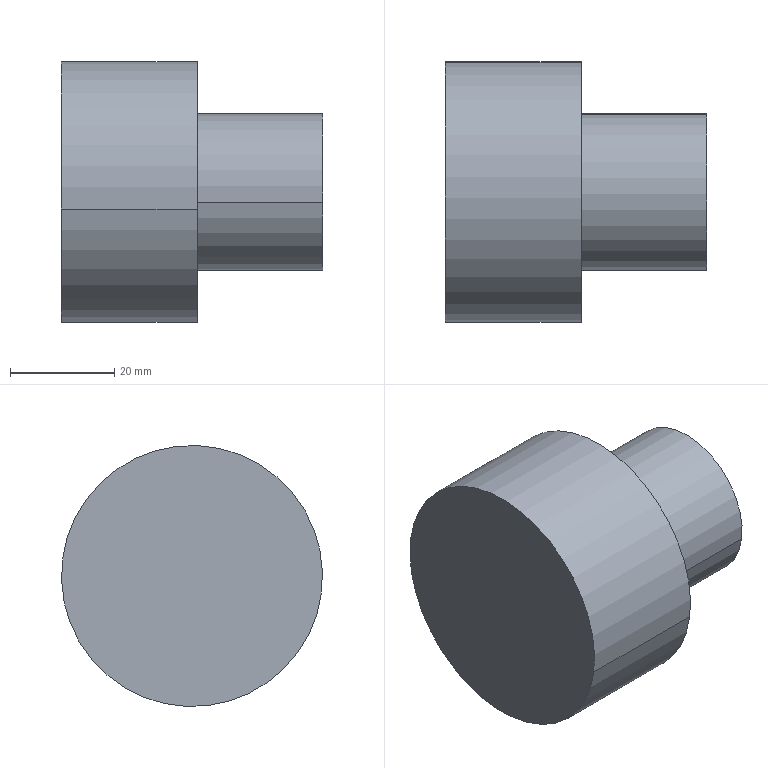Component | SolidWorks | -BeltTensionHandwheel-1 | 1 solid | 10 faces | box 50 x 50 x 50 mm | volume 66319 mm3 | cylinder 6 | plane 4 | commonest cylinder face diameters 12 x2 30 x2 50 x2
build123d program:
from build123d import *


with BuildPart() as part:
    # Sketch1 → Revolve1 (revolve)
    with BuildSketch(Plane.XY):
        Polygon((0, 0), (25, 0), (25, 26), (15, 26), (15, 50), (6, 50), (6, 35), (0, 35), align=None)
    revolve(axis=Axis((0, -469.095, 0), (0, 1, 0)))


solid = part.part

# Placed as in the assembly
solid = solid.moved(Location((-325, 1094.5, -20), (0, 0, -90)))
STEP:
#1=COLOUR_RGB('',0.7922,0.8196,0.9333);
#2=FILL_AREA_STYLE_COLOUR('',#1);
#3=FILL_AREA_STYLE('',(#2));
#4=SURFACE_STYLE_FILL_AREA(#3);
#5=SURFACE_SIDE_STYLE('',(#4));
#6=SURFACE_STYLE_USAGE(.BOTH.,#5);
#7=PRESENTATION_STYLE_ASSIGNMENT((#6));
#8=CARTESIAN_POINT('',(-10.827,43.325,-0.7566));
#9=VERTEX_POINT('',#8);
#10=CARTESIAN_POINT('',(-10.827,42.856,-0.8182));
#11=VERTEX_POINT('',#10);
#12=CARTESIAN_POINT('',(-10.827,43.091,-0.7874));
#13=DIRECTION('',(-1.,0.,-0.));
#14=DIRECTION('',(-0.,-0.9915,-0.1304));
#15=AXIS2_PLACEMENT_3D('',#12,#13,#14);
#16=CIRCLE('',#15,0.2362);
#17=EDGE_CURVE('',#9,#11,#16,.T.);
#18=ORIENTED_EDGE('',*,*,#17,.F.);
#19=CARTESIAN_POINT('',(-11.417,43.325,-0.7566));
#20=VERTEX_POINT('',#19);
#21=CARTESIAN_POINT('',(-31.264,43.325,-0.7566));
#22=DIRECTION('',(-1.,0.,-0.));
#23=VECTOR('',#22,39.37);
#24=LINE('',#21,#23);
#25=EDGE_CURVE('',#9,#20,#24,.T.);
#26=ORIENTED_EDGE('',*,*,#25,.T.);
#27=CARTESIAN_POINT('',(-11.417,42.856,-0.8182));
#28=VERTEX_POINT('',#27);
#29=CARTESIAN_POINT('',(-11.417,43.091,-0.7874));
#30=DIRECTION('',(-1.,0.,-0.));
#31=DIRECTION('',(-0.,-0.9915,-0.1304));
#32=AXIS2_PLACEMENT_3D('',#29,#30,#31);
#33=CIRCLE('',#32,0.2362);
#34=EDGE_CURVE('',#20,#28,#33,.T.);
#35=ORIENTED_EDGE('',*,*,#34,.T.);
#36=CARTESIAN_POINT('',(-31.264,42.856,-0.8182));
#37=DIRECTION('',(-1.,0.,-0.));
#38=VECTOR('',#37,39.37);
#39=LINE('',#36,#38);
#40=EDGE_CURVE('',#11,#28,#39,.T.);
#41=ORIENTED_EDGE('',*,*,#40,.F.);
#42=EDGE_LOOP('',(#18,#26,#35,#41));
#43=FACE_OUTER_BOUND('',#42,.T.);
#44=CARTESIAN_POINT('',(-31.264,43.091,-0.7874));
#45=DIRECTION('',(-1.,0.,-0.));
#46=DIRECTION('',(-0.,-0.9915,-0.1304));
#47=AXIS2_PLACEMENT_3D('',#44,#45,#46);
#48=CYLINDRICAL_SURFACE('',#47,0.2362);
#49=ADVANCED_FACE('',(#43),#48,.F.);
#50=CARTESIAN_POINT('',(-10.827,42.505,-0.8644));
#51=VERTEX_POINT('',#50);
#52=CARTESIAN_POINT('',(-10.827,43.676,-0.7104));
#53=VERTEX_POINT('',#52);
#54=CARTESIAN_POINT('',(-10.827,43.091,-0.7874));
#55=DIRECTION('',(-1.,0.,-0.));
#56=DIRECTION('',(-0.,-0.9915,-0.1304));
#57=AXIS2_PLACEMENT_3D('',#54,#55,#56);
#58=CIRCLE('',#57,0.5906);
#59=EDGE_CURVE('',#51,#53,#58,.T.);
#60=ORIENTED_EDGE('',*,*,#59,.T.);
#61=CARTESIAN_POINT('',(-11.772,43.676,-0.7104));
#62=VERTEX_POINT('',#61);
#63=CARTESIAN_POINT('',(-31.264,43.676,-0.7104));
#64=DIRECTION('',(-1.,0.,-0.));
#65=VECTOR('',#64,39.37);
#66=LINE('',#63,#65);
#67=EDGE_CURVE('',#53,#62,#66,.T.);
#68=ORIENTED_EDGE('',*,*,#67,.T.);
#69=CARTESIAN_POINT('',(-11.772,42.505,-0.8644));
#70=VERTEX_POINT('',#69);
#71=CARTESIAN_POINT('',(-11.772,43.091,-0.7874));
#72=DIRECTION('',(-1.,0.,-0.));
#73=DIRECTION('',(-0.,-0.9915,-0.1304));
#74=AXIS2_PLACEMENT_3D('',#71,#72,#73);
#75=CIRCLE('',#74,0.5906);
#76=EDGE_CURVE('',#70,#62,#75,.T.);
#77=ORIENTED_EDGE('',*,*,#76,.F.);
#78=CARTESIAN_POINT('',(-31.264,42.505,-0.8644));
#79=DIRECTION('',(-1.,0.,-0.));
#80=VECTOR('',#79,39.37);
#81=LINE('',#78,#80);
#82=EDGE_CURVE('',#51,#70,#81,.T.);
#83=ORIENTED_EDGE('',*,*,#82,.F.);
#84=EDGE_LOOP('',(#60,#68,#77,#83));
#85=FACE_OUTER_BOUND('',#84,.T.);
#86=CARTESIAN_POINT('',(-31.264,43.091,-0.7874));
#87=DIRECTION('',(-1.,0.,-0.));
#88=DIRECTION('',(-0.,-0.9915,-0.1304));
#89=AXIS2_PLACEMENT_3D('',#86,#87,#88);
#90=CYLINDRICAL_SURFACE('',#89,0.5906);
#91=ADVANCED_FACE('',(#85),#90,.T.);
#92=CARTESIAN_POINT('',(-11.772,42.115,-0.9158));
#93=VERTEX_POINT('',#92);
#94=CARTESIAN_POINT('',(-11.772,44.066,-0.659));
#95=VERTEX_POINT('',#94);
#96=CARTESIAN_POINT('',(-11.772,43.091,-0.7874));
#97=DIRECTION('',(-1.,0.,-0.));
#98=DIRECTION('',(-0.,-0.9915,-0.1304));
#99=AXIS2_PLACEMENT_3D('',#96,#97,#98);
#100=CIRCLE('',#99,0.9843);
#101=EDGE_CURVE('',#93,#95,#100,.T.);
#102=ORIENTED_EDGE('',*,*,#101,.T.);
#103=CARTESIAN_POINT('',(-12.795,44.066,-0.659));
#104=VERTEX_POINT('',#103);
#105=CARTESIAN_POINT('',(-31.264,44.066,-0.659));
#106=DIRECTION('',(-1.,0.,-0.));
#107=VECTOR('',#106,39.37);
#108=LINE('',#105,#107);
#109=EDGE_CURVE('',#95,#104,#108,.T.);
#110=ORIENTED_EDGE('',*,*,#109,.T.);
#111=CARTESIAN_POINT('',(-12.795,42.115,-0.9158));
#112=VERTEX_POINT('',#111);
#113=CARTESIAN_POINT('',(-12.795,43.091,-0.7874));
#114=DIRECTION('',(-1.,0.,-0.));
#115=DIRECTION('',(-0.,-0.9915,-0.1304));
#116=AXIS2_PLACEMENT_3D('',#113,#114,#115);
#117=CIRCLE('',#116,0.9843);
#118=EDGE_CURVE('',#112,#104,#117,.T.);
#119=ORIENTED_EDGE('',*,*,#118,.F.);
#120=CARTESIAN_POINT('',(-31.264,42.115,-0.9158));
#121=DIRECTION('',(-1.,0.,-0.));
#122=VECTOR('',#121,39.37);
#123=LINE('',#120,#122);
#124=EDGE_CURVE('',#93,#112,#123,.T.);
#125=ORIENTED_EDGE('',*,*,#124,.F.);
#126=EDGE_LOOP('',(#102,#110,#119,#125));
#127=FACE_OUTER_BOUND('',#126,.T.);
#128=CARTESIAN_POINT('',(-31.264,43.091,-0.7874));
#129=DIRECTION('',(-1.,0.,-0.));
#130=DIRECTION('',(-0.,-0.9915,-0.1304));
#131=AXIS2_PLACEMENT_3D('',#128,#129,#130);
#132=CYLINDRICAL_SURFACE('',#131,0.9843);
#133=ADVANCED_FACE('',(#127),#132,.T.);
#134=ORIENTED_EDGE('',*,*,#118,.T.);
#135=CARTESIAN_POINT('',(-12.795,43.091,-0.7874));
#136=DIRECTION('',(-1.,0.,-0.));
#137=DIRECTION('',(-0.,-0.9915,-0.1304));
#138=AXIS2_PLACEMENT_3D('',#135,#136,#137);
#139=CIRCLE('',#138,0.9843);
#140=EDGE_CURVE('',#104,#112,#139,.T.);
#141=ORIENTED_EDGE('',*,*,#140,.T.);
#142=EDGE_LOOP('',(#134,#141));
#143=FACE_OUTER_BOUND('',#142,.T.);
#144=CARTESIAN_POINT('',(-12.795,43.091,-0.7874));
#145=DIRECTION('',(-1.,0.,-0.));
#146=DIRECTION('',(-0.,-0.9915,-0.1304));
#147=AXIS2_PLACEMENT_3D('',#144,#145,#146);
#148=PLANE('',#147);
#149=ADVANCED_FACE('',(#143),#148,.T.);
#150=ORIENTED_EDGE('',*,*,#109,.F.);
#151=CARTESIAN_POINT('',(-11.772,43.091,-0.7874));
#152=DIRECTION('',(-1.,0.,-0.));
#153=DIRECTION('',(-0.,-0.9915,-0.1304));
#154=AXIS2_PLACEMENT_3D('',#151,#152,#153);
#155=CIRCLE('',#154,0.9843);
#156=EDGE_CURVE('',#95,#93,#155,.T.);
#157=ORIENTED_EDGE('',*,*,#156,.T.);
#158=ORIENTED_EDGE('',*,*,#124,.T.);
#159=ORIENTED_EDGE('',*,*,#140,.F.);
#160=EDGE_LOOP('',(#150,#157,#158,#159));
#161=FACE_OUTER_BOUND('',#160,.T.);
#162=CARTESIAN_POINT('',(-31.264,43.091,-0.7874));
#163=DIRECTION('',(-1.,0.,-0.));
#164=DIRECTION('',(-0.,-0.9915,-0.1304));
#165=AXIS2_PLACEMENT_3D('',#162,#163,#164);
#166=CYLINDRICAL_SURFACE('',#165,0.9843);
#167=ADVANCED_FACE('',(#161),#166,.T.);
#168=ORIENTED_EDGE('',*,*,#76,.T.);
#169=CARTESIAN_POINT('',(-11.772,43.091,-0.7874));
#170=DIRECTION('',(-1.,0.,-0.));
#171=DIRECTION('',(-0.,-0.9915,-0.1304));
#172=AXIS2_PLACEMENT_3D('',#169,#170,#171);
#173=CIRCLE('',#172,0.5906);
#174=EDGE_CURVE('',#62,#70,#173,.T.);
#175=ORIENTED_EDGE('',*,*,#174,.T.);
#176=EDGE_LOOP('',(#168,#175));
#177=FACE_BOUND('',#176,.T.);
#178=ORIENTED_EDGE('',*,*,#101,.F.);
#179=ORIENTED_EDGE('',*,*,#156,.F.);
#180=EDGE_LOOP('',(#178,#179));
#181=FACE_OUTER_BOUND('',#180,.T.);
#182=CARTESIAN_POINT('',(-11.772,42.115,-0.9158));
#183=DIRECTION('',(1.,-0.,0.));
#184=DIRECTION('',(0.,0.9915,0.1304));
#185=AXIS2_PLACEMENT_3D('',#182,#183,#184);
#186=PLANE('',#185);
#187=ADVANCED_FACE('',(#177,#181),#186,.T.);
#188=ORIENTED_EDGE('',*,*,#67,.F.);
#189=CARTESIAN_POINT('',(-10.827,43.091,-0.7874));
#190=DIRECTION('',(-1.,0.,-0.));
#191=DIRECTION('',(-0.,-0.9915,-0.1304));
#192=AXIS2_PLACEMENT_3D('',#189,#190,#191);
#193=CIRCLE('',#192,0.5906);
#194=EDGE_CURVE('',#53,#51,#193,.T.);
#195=ORIENTED_EDGE('',*,*,#194,.T.);
#196=ORIENTED_EDGE('',*,*,#82,.T.);
#197=ORIENTED_EDGE('',*,*,#174,.F.);
#198=EDGE_LOOP('',(#188,#195,#196,#197));
#199=FACE_OUTER_BOUND('',#198,.T.);
#200=CARTESIAN_POINT('',(-31.264,43.091,-0.7874));
#201=DIRECTION('',(-1.,0.,-0.));
#202=DIRECTION('',(-0.,-0.9915,-0.1304));
#203=AXIS2_PLACEMENT_3D('',#200,#201,#202);
#204=CYLINDRICAL_SURFACE('',#203,0.5906);
#205=ADVANCED_FACE('',(#199),#204,.T.);
#206=CARTESIAN_POINT('',(-10.827,43.091,-0.7874));
#207=DIRECTION('',(-1.,0.,-0.));
#208=DIRECTION('',(-0.,-0.9915,-0.1304));
#209=AXIS2_PLACEMENT_3D('',#206,#207,#208);
#210=CIRCLE('',#209,0.2362);
#211=EDGE_CURVE('',#11,#9,#210,.T.);
#212=ORIENTED_EDGE('',*,*,#211,.T.);
#213=ORIENTED_EDGE('',*,*,#17,.T.);
#214=EDGE_LOOP('',(#212,#213));
#215=FACE_BOUND('',#214,.T.);
#216=ORIENTED_EDGE('',*,*,#59,.F.);
#217=ORIENTED_EDGE('',*,*,#194,.F.);
#218=EDGE_LOOP('',(#216,#217));
#219=FACE_OUTER_BOUND('',#218,.T.);
#220=CARTESIAN_POINT('',(-10.827,42.505,-0.8644));
#221=DIRECTION('',(1.,-0.,0.));
#222=DIRECTION('',(0.,0.9915,0.1304));
#223=AXIS2_PLACEMENT_3D('',#220,#221,#222);
#224=PLANE('',#223);
#225=ADVANCED_FACE('',(#215,#219),#224,.T.);
#226=ORIENTED_EDGE('',*,*,#25,.F.);
#227=ORIENTED_EDGE('',*,*,#211,.F.);
#228=ORIENTED_EDGE('',*,*,#40,.T.);
#229=CARTESIAN_POINT('',(-11.417,43.091,-0.7874));
#230=DIRECTION('',(-1.,0.,-0.));
#231=DIRECTION('',(-0.,-0.9915,-0.1304));
#232=AXIS2_PLACEMENT_3D('',#229,#230,#231);
#233=CIRCLE('',#232,0.2362);
#234=EDGE_CURVE('',#28,#20,#233,.T.);
#235=ORIENTED_EDGE('',*,*,#234,.T.);
#236=EDGE_LOOP('',(#226,#227,#228,#235));
#237=FACE_OUTER_BOUND('',#236,.T.);
#238=CARTESIAN_POINT('',(-31.264,43.091,-0.7874));
#239=DIRECTION('',(-1.,0.,-0.));
#240=DIRECTION('',(-0.,-0.9915,-0.1304));
#241=AXIS2_PLACEMENT_3D('',#238,#239,#240);
#242=CYLINDRICAL_SURFACE('',#241,0.2362);
#243=ADVANCED_FACE('',(#237),#242,.F.);
#244=ORIENTED_EDGE('',*,*,#234,.F.);
#245=ORIENTED_EDGE('',*,*,#34,.F.);
#246=EDGE_LOOP('',(#244,#245));
#247=FACE_OUTER_BOUND('',#246,.T.);
#248=CARTESIAN_POINT('',(-11.417,42.856,-0.8182));
#249=DIRECTION('',(1.,-0.,0.));
#250=DIRECTION('',(0.,0.9915,0.1304));
#251=AXIS2_PLACEMENT_3D('',#248,#249,#250);
#252=PLANE('',#251);
#253=ADVANCED_FACE('',(#247),#252,.T.);
#254=CLOSED_SHELL('',(#49,#91,#133,#149,#167,#187,#205,#225,#243,#253));
#255=MANIFOLD_SOLID_BREP('',#254);
#256=STYLED_ITEM('',(#7),#255);
#257=PRESENTATION_LAYER_ASSIGNMENT('','',(#256));
#258=(LENGTH_UNIT()NAMED_UNIT(*)SI_UNIT($,.METRE.));
#259=LENGTH_MEASURE_WITH_UNIT(LENGTH_MEASURE(0.0254),#258);
#260=DIMENSIONAL_EXPONENTS(1.,0.,0.,0.,0.,0.,0.);
#261=(CONVERSION_BASED_UNIT('',#259)LENGTH_UNIT()NAMED_UNIT(#260));
#262=UNCERTAINTY_MEASURE_WITH_UNIT(LENGTH_MEASURE(0.00001),#261,'','');
#263=(NAMED_UNIT(*)PLANE_ANGLE_UNIT()SI_UNIT($,.RADIAN.));
#264=(NAMED_UNIT(*)SI_UNIT($,.STERADIAN.)SOLID_ANGLE_UNIT());
#265=(GEOMETRIC_REPRESENTATION_CONTEXT(3)GLOBAL_UNCERTAINTY_ASSIGNED_CONTEXT((#262))GLOBAL_UNIT_ASSIGNED_CONTEXT((#261,#263,#264))REPRESENTATION_CONTEXT('',''));
#266=MECHANICAL_DESIGN_GEOMETRIC_PRESENTATION_REPRESENTATION('',(#256),#265);
#267=CARTESIAN_POINT('',(0.,0.,0.));
#268=DIRECTION('',(0.,0.,1.));
#269=DIRECTION('',(1.,0.,0.));
#270=AXIS2_PLACEMENT_3D('',#267,#268,#269);
#271=(LENGTH_UNIT()NAMED_UNIT(*)SI_UNIT($,.METRE.));
#272=LENGTH_MEASURE_WITH_UNIT(LENGTH_MEASURE(0.0254),#271);
#273=DIMENSIONAL_EXPONENTS(1.,0.,0.,0.,0.,0.,0.);
#274=(CONVERSION_BASED_UNIT('',#272)LENGTH_UNIT()NAMED_UNIT(#273));
#275=UNCERTAINTY_MEASURE_WITH_UNIT(LENGTH_MEASURE(0.00001),#274,'','');
#276=(NAMED_UNIT(*)PLANE_ANGLE_UNIT()SI_UNIT($,.RADIAN.));
#277=(NAMED_UNIT(*)SI_UNIT($,.STERADIAN.)SOLID_ANGLE_UNIT());
#278=(GEOMETRIC_REPRESENTATION_CONTEXT(3)GLOBAL_UNCERTAINTY_ASSIGNED_CONTEXT((#275))GLOBAL_UNIT_ASSIGNED_CONTEXT((#274,#276,#277))REPRESENTATION_CONTEXT('',''));
#279=ADVANCED_BREP_SHAPE_REPRESENTATION('',(#255,#270),#278);